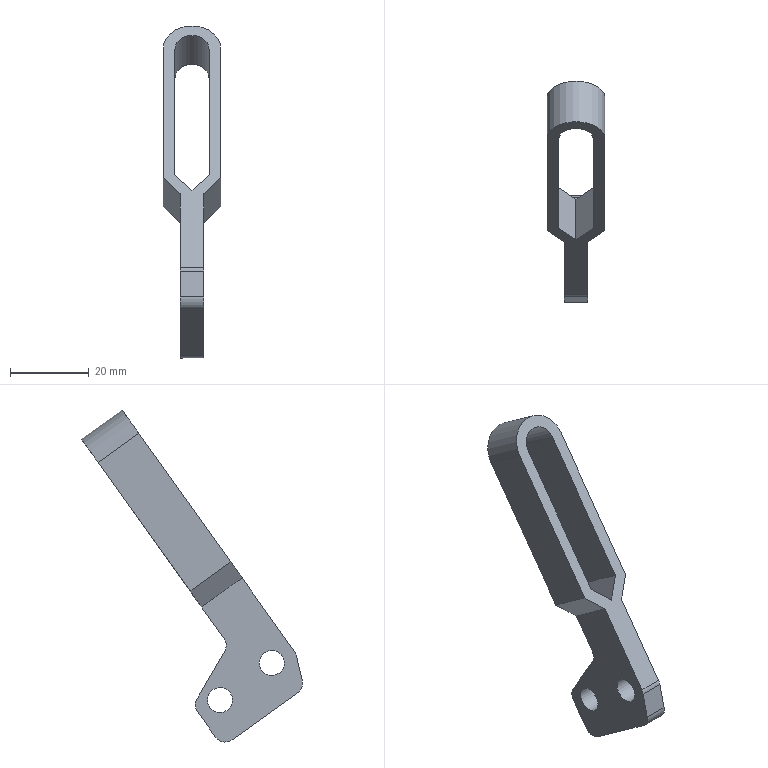Component | SolidWorks | AD12-MC01H-4_2_03.SDASM-1_AD12-_MC01H-4_s.sdprt-1 | 1 solid | 27 faces | box 14.7 x 56.22 x 84.43 mm | volume 7823 mm3 | plane 16 | cylinder 11 | commonest cylinder face diameters 6 x5 6.35 x4 14.7 x1 8.7 x1
STEP:
#1=COLOUR_RGB('',0.7922,0.8196,0.9333);
#2=FILL_AREA_STYLE_COLOUR('',#1);
#3=FILL_AREA_STYLE('',(#2));
#4=SURFACE_STYLE_FILL_AREA(#3);
#5=SURFACE_SIDE_STYLE('',(#4));
#6=SURFACE_STYLE_USAGE(.BOTH.,#5);
#7=PRESENTATION_STYLE_ASSIGNMENT((#6));
#8=CARTESIAN_POINT('',(-12.398,-8.023,13.819));
#9=VERTEX_POINT('',#8);
#10=CARTESIAN_POINT('',(-12.398,-8.168,13.616));
#11=VERTEX_POINT('',#10);
#12=CARTESIAN_POINT('',(-12.398,-8.096,13.717));
#13=DIRECTION('',(1.,0.,0.));
#14=DIRECTION('',(0.,-0.5813,-0.8137));
#15=AXIS2_PLACEMENT_3D('',#12,#13,#14);
#16=CIRCLE('',#15,0.125);
#17=EDGE_CURVE('',#9,#11,#16,.T.);
#18=ORIENTED_EDGE('',*,*,#17,.F.);
#19=CARTESIAN_POINT('',(-12.162,-8.023,13.819));
#20=VERTEX_POINT('',#19);
#21=CARTESIAN_POINT('',(-12.398,-8.023,13.819));
#22=DIRECTION('',(1.,0.,0.));
#23=VECTOR('',#22,39.37);
#24=LINE('',#21,#23);
#25=EDGE_CURVE('',#9,#20,#24,.T.);
#26=ORIENTED_EDGE('',*,*,#25,.T.);
#27=CARTESIAN_POINT('',(-12.162,-8.168,13.616));
#28=VERTEX_POINT('',#27);
#29=CARTESIAN_POINT('',(-12.162,-8.096,13.717));
#30=DIRECTION('',(1.,0.,0.));
#31=DIRECTION('',(0.,-0.5813,-0.8137));
#32=AXIS2_PLACEMENT_3D('',#29,#30,#31);
#33=CIRCLE('',#32,0.125);
#34=EDGE_CURVE('',#20,#28,#33,.T.);
#35=ORIENTED_EDGE('',*,*,#34,.T.);
#36=CARTESIAN_POINT('',(-12.398,-8.168,13.616));
#37=DIRECTION('',(1.,0.,0.));
#38=VECTOR('',#37,39.37);
#39=LINE('',#36,#38);
#40=EDGE_CURVE('',#11,#28,#39,.T.);
#41=ORIENTED_EDGE('',*,*,#40,.F.);
#42=EDGE_LOOP('',(#18,#26,#35,#41));
#43=FACE_OUTER_BOUND('',#42,.T.);
#44=CARTESIAN_POINT('',(-12.398,-8.096,13.717));
#45=DIRECTION('',(1.,0.,0.));
#46=DIRECTION('',(0.,-0.5813,-0.8137));
#47=AXIS2_PLACEMENT_3D('',#44,#45,#46);
#48=CYLINDRICAL_SURFACE('',#47,0.125);
#49=ADVANCED_FACE('',(#43),#48,.F.);
#50=CARTESIAN_POINT('',(-12.398,-8.542,14.19));
#51=VERTEX_POINT('',#50);
#52=CARTESIAN_POINT('',(-12.398,-8.687,13.986));
#53=VERTEX_POINT('',#52);
#54=CARTESIAN_POINT('',(-12.398,-8.615,14.088));
#55=DIRECTION('',(1.,0.,0.));
#56=DIRECTION('',(0.,-0.5813,-0.8137));
#57=AXIS2_PLACEMENT_3D('',#54,#55,#56);
#58=CIRCLE('',#57,0.125);
#59=EDGE_CURVE('',#51,#53,#58,.T.);
#60=ORIENTED_EDGE('',*,*,#59,.F.);
#61=CARTESIAN_POINT('',(-12.162,-8.542,14.19));
#62=VERTEX_POINT('',#61);
#63=CARTESIAN_POINT('',(-12.398,-8.542,14.19));
#64=DIRECTION('',(1.,0.,0.));
#65=VECTOR('',#64,39.37);
#66=LINE('',#63,#65);
#67=EDGE_CURVE('',#51,#62,#66,.T.);
#68=ORIENTED_EDGE('',*,*,#67,.T.);
#69=CARTESIAN_POINT('',(-12.162,-8.687,13.986));
#70=VERTEX_POINT('',#69);
#71=CARTESIAN_POINT('',(-12.162,-8.615,14.088));
#72=DIRECTION('',(1.,0.,0.));
#73=DIRECTION('',(0.,-0.5813,-0.8137));
#74=AXIS2_PLACEMENT_3D('',#71,#72,#73);
#75=CIRCLE('',#74,0.125);
#76=EDGE_CURVE('',#62,#70,#75,.T.);
#77=ORIENTED_EDGE('',*,*,#76,.T.);
#78=CARTESIAN_POINT('',(-12.398,-8.687,13.986));
#79=DIRECTION('',(1.,0.,0.));
#80=VECTOR('',#79,39.37);
#81=LINE('',#78,#80);
#82=EDGE_CURVE('',#53,#70,#81,.T.);
#83=ORIENTED_EDGE('',*,*,#82,.F.);
#84=EDGE_LOOP('',(#60,#68,#77,#83));
#85=FACE_OUTER_BOUND('',#84,.T.);
#86=CARTESIAN_POINT('',(-12.398,-8.615,14.088));
#87=DIRECTION('',(1.,0.,0.));
#88=DIRECTION('',(0.,-0.5813,-0.8137));
#89=AXIS2_PLACEMENT_3D('',#86,#87,#88);
#90=CYLINDRICAL_SURFACE('',#89,0.125);
#91=ADVANCED_FACE('',(#85),#90,.F.);
#92=CARTESIAN_POINT('',(-12.162,-8.096,13.717));
#93=DIRECTION('',(1.,0.,0.));
#94=DIRECTION('',(0.,-0.5813,-0.8137));
#95=AXIS2_PLACEMENT_3D('',#92,#93,#94);
#96=CIRCLE('',#95,0.125);
#97=EDGE_CURVE('',#28,#20,#96,.T.);
#98=ORIENTED_EDGE('',*,*,#97,.F.);
#99=ORIENTED_EDGE('',*,*,#34,.F.);
#100=EDGE_LOOP('',(#98,#99));
#101=FACE_BOUND('',#100,.T.);
#102=CARTESIAN_POINT('',(-12.162,-7.91,14.648));
#103=VERTEX_POINT('',#102);
#104=CARTESIAN_POINT('',(-12.162,-8.136,14.331));
#105=VERTEX_POINT('',#104);
#106=CARTESIAN_POINT('',(-12.162,-7.91,14.648));
#107=DIRECTION('',(0.,-0.5813,-0.8137));
#108=VECTOR('',#107,39.37);
#109=LINE('',#106,#108);
#110=EDGE_CURVE('',#103,#105,#109,.T.);
#111=ORIENTED_EDGE('',*,*,#110,.F.);
#112=CARTESIAN_POINT('',(-12.162,-8.316,14.939));
#113=VERTEX_POINT('',#112);
#114=CARTESIAN_POINT('',(-12.162,-7.195,14.138));
#115=DIRECTION('',(0.,0.8137,-0.5813));
#116=VECTOR('',#115,39.37);
#117=LINE('',#114,#116);
#118=EDGE_CURVE('',#113,#103,#117,.T.);
#119=ORIENTED_EDGE('',*,*,#118,.F.);
#120=CARTESIAN_POINT('',(-12.162,-8.84,14.206));
#121=VERTEX_POINT('',#120);
#122=CARTESIAN_POINT('',(-12.162,-8.316,14.939));
#123=DIRECTION('',(0.,0.5813,0.8137));
#124=VECTOR('',#123,39.37);
#125=LINE('',#122,#124);
#126=EDGE_CURVE('',#121,#113,#125,.T.);
#127=ORIENTED_EDGE('',*,*,#126,.F.);
#128=CARTESIAN_POINT('',(-12.162,-8.859,14.164));
#129=VERTEX_POINT('',#128);
#130=CARTESIAN_POINT('',(-12.162,-8.744,14.137));
#131=DIRECTION('',(-1.,0.,0.));
#132=DIRECTION('',(0.,-0.5813,-0.8137));
#133=AXIS2_PLACEMENT_3D('',#130,#131,#132);
#134=CIRCLE('',#133,0.1181);
#135=EDGE_CURVE('',#129,#121,#134,.T.);
#136=ORIENTED_EDGE('',*,*,#135,.F.);
#137=CARTESIAN_POINT('',(-12.162,-8.918,13.911));
#138=VERTEX_POINT('',#137);
#139=CARTESIAN_POINT('',(-12.162,-8.918,13.911));
#140=DIRECTION('',(0.,0.2274,0.9738));
#141=VECTOR('',#140,39.37);
#142=LINE('',#139,#141);
#143=EDGE_CURVE('',#138,#129,#142,.T.);
#144=ORIENTED_EDGE('',*,*,#143,.F.);
#145=CARTESIAN_POINT('',(-12.162,-8.872,13.788));
#146=VERTEX_POINT('',#145);
#147=CARTESIAN_POINT('',(-12.162,-8.803,13.884));
#148=DIRECTION('',(-1.,0.,0.));
#149=DIRECTION('',(0.,-0.5813,-0.8137));
#150=AXIS2_PLACEMENT_3D('',#147,#148,#149);
#151=CIRCLE('',#150,0.1181);
#152=EDGE_CURVE('',#146,#138,#151,.T.);
#153=ORIENTED_EDGE('',*,*,#152,.F.);
#154=CARTESIAN_POINT('',(-12.162,-8.216,13.319));
#155=VERTEX_POINT('',#154);
#156=CARTESIAN_POINT('',(-12.162,-7.927,13.113));
#157=DIRECTION('',(0.,-0.8137,0.5813));
#158=VECTOR('',#157,39.37);
#159=LINE('',#156,#158);
#160=EDGE_CURVE('',#155,#146,#159,.T.);
#161=ORIENTED_EDGE('',*,*,#160,.F.);
#162=CARTESIAN_POINT('',(-12.162,-8.051,13.347));
#163=VERTEX_POINT('',#162);
#164=CARTESIAN_POINT('',(-12.162,-8.147,13.415));
#165=DIRECTION('',(-1.,0.,0.));
#166=DIRECTION('',(0.,-0.5813,-0.8137));
#167=AXIS2_PLACEMENT_3D('',#164,#165,#166);
#168=CIRCLE('',#167,0.1181);
#169=EDGE_CURVE('',#163,#155,#168,.T.);
#170=ORIENTED_EDGE('',*,*,#169,.F.);
#171=CARTESIAN_POINT('',(-12.162,-7.87,13.599));
#172=VERTEX_POINT('',#171);
#173=CARTESIAN_POINT('',(-12.162,-7.387,14.275));
#174=DIRECTION('',(0.,-0.5813,-0.8137));
#175=VECTOR('',#174,39.37);
#176=LINE('',#173,#175);
#177=EDGE_CURVE('',#172,#163,#176,.T.);
#178=ORIENTED_EDGE('',*,*,#177,.F.);
#179=CARTESIAN_POINT('',(-12.162,-7.865,13.727));
#180=VERTEX_POINT('',#179);
#181=CARTESIAN_POINT('',(-12.162,-7.967,13.668));
#182=DIRECTION('',(-1.,0.,0.));
#183=DIRECTION('',(0.,-0.5813,-0.8137));
#184=AXIS2_PLACEMENT_3D('',#181,#182,#183);
#185=CIRCLE('',#184,0.1181);
#186=EDGE_CURVE('',#180,#172,#185,.T.);
#187=ORIENTED_EDGE('',*,*,#186,.F.);
#188=CARTESIAN_POINT('',(-12.162,-8.142,14.203));
#189=VERTEX_POINT('',#188);
#190=CARTESIAN_POINT('',(-12.162,-8.142,14.203));
#191=DIRECTION('',(0.,0.5037,-0.8639));
#192=VECTOR('',#191,39.37);
#193=LINE('',#190,#192);
#194=EDGE_CURVE('',#189,#180,#193,.T.);
#195=ORIENTED_EDGE('',*,*,#194,.F.);
#196=CARTESIAN_POINT('',(-12.162,-8.04,14.263));
#197=DIRECTION('',(1.,0.,0.));
#198=DIRECTION('',(0.,-0.5813,-0.8137));
#199=AXIS2_PLACEMENT_3D('',#196,#197,#198);
#200=CIRCLE('',#199,0.1181);
#201=EDGE_CURVE('',#105,#189,#200,.T.);
#202=ORIENTED_EDGE('',*,*,#201,.F.);
#203=EDGE_LOOP('',(#111,#119,#127,#136,#144,#153,#161,#170,#178,#187,#195,#202));
#204=FACE_OUTER_BOUND('',#203,.T.);
#205=CARTESIAN_POINT('',(-12.162,-8.615,14.088));
#206=DIRECTION('',(1.,0.,0.));
#207=DIRECTION('',(0.,-0.5813,-0.8137));
#208=AXIS2_PLACEMENT_3D('',#205,#206,#207);
#209=CIRCLE('',#208,0.125);
#210=EDGE_CURVE('',#70,#62,#209,.T.);
#211=ORIENTED_EDGE('',*,*,#210,.F.);
#212=ORIENTED_EDGE('',*,*,#76,.F.);
#213=EDGE_LOOP('',(#211,#212));
#214=FACE_BOUND('',#213,.T.);
#215=CARTESIAN_POINT('',(-12.162,-7.195,14.138));
#216=DIRECTION('',(-1.,0.,0.));
#217=DIRECTION('',(0.,0.5813,0.8137));
#218=AXIS2_PLACEMENT_3D('',#215,#216,#217);
#219=PLANE('',#218);
#220=ADVANCED_FACE('',(#101,#204,#214),#219,.F.);
#221=ORIENTED_EDGE('',*,*,#25,.F.);
#222=CARTESIAN_POINT('',(-12.398,-8.096,13.717));
#223=DIRECTION('',(1.,0.,0.));
#224=DIRECTION('',(0.,-0.5813,-0.8137));
#225=AXIS2_PLACEMENT_3D('',#222,#223,#224);
#226=CIRCLE('',#225,0.125);
#227=EDGE_CURVE('',#11,#9,#226,.T.);
#228=ORIENTED_EDGE('',*,*,#227,.F.);
#229=ORIENTED_EDGE('',*,*,#40,.T.);
#230=ORIENTED_EDGE('',*,*,#97,.T.);
#231=EDGE_LOOP('',(#221,#228,#229,#230));
#232=FACE_OUTER_BOUND('',#231,.T.);
#233=CARTESIAN_POINT('',(-12.398,-8.096,13.717));
#234=DIRECTION('',(1.,0.,0.));
#235=DIRECTION('',(0.,-0.5813,-0.8137));
#236=AXIS2_PLACEMENT_3D('',#233,#234,#235);
#237=CYLINDRICAL_SURFACE('',#236,0.125);
#238=ADVANCED_FACE('',(#232),#237,.F.);
#239=CARTESIAN_POINT('',(-12.398,-8.142,14.203));
#240=VERTEX_POINT('',#239);
#241=CARTESIAN_POINT('',(-10.902,-8.142,14.203));
#242=DIRECTION('',(1.,0.,0.));
#243=VECTOR('',#242,39.37);
#244=LINE('',#241,#243);
#245=EDGE_CURVE('',#240,#189,#244,.T.);
#246=ORIENTED_EDGE('',*,*,#245,.F.);
#247=CARTESIAN_POINT('',(-12.398,-8.136,14.331));
#248=VERTEX_POINT('',#247);
#249=CARTESIAN_POINT('',(-12.398,-8.04,14.263));
#250=DIRECTION('',(1.,0.,0.));
#251=DIRECTION('',(0.,-0.5813,-0.8137));
#252=AXIS2_PLACEMENT_3D('',#249,#250,#251);
#253=CIRCLE('',#252,0.1181);
#254=EDGE_CURVE('',#248,#240,#253,.T.);
#255=ORIENTED_EDGE('',*,*,#254,.F.);
#256=CARTESIAN_POINT('',(-10.902,-8.136,14.331));
#257=DIRECTION('',(-1.,0.,0.));
#258=VECTOR('',#257,39.37);
#259=LINE('',#256,#258);
#260=EDGE_CURVE('',#105,#248,#259,.T.);
#261=ORIENTED_EDGE('',*,*,#260,.F.);
#262=ORIENTED_EDGE('',*,*,#201,.T.);
#263=EDGE_LOOP('',(#246,#255,#261,#262));
#264=FACE_OUTER_BOUND('',#263,.T.);
#265=CARTESIAN_POINT('',(-10.902,-8.04,14.263));
#266=DIRECTION('',(1.,0.,0.));
#267=DIRECTION('',(0.,-0.5813,-0.8137));
#268=AXIS2_PLACEMENT_3D('',#265,#266,#267);
#269=CYLINDRICAL_SURFACE('',#268,0.1181);
#270=ADVANCED_FACE('',(#264),#269,.F.);
#271=CARTESIAN_POINT('',(-12.398,-7.91,14.648));
#272=VERTEX_POINT('',#271);
#273=CARTESIAN_POINT('',(-12.398,-8.136,14.331));
#274=DIRECTION('',(0.,-0.5813,-0.8137));
#275=VECTOR('',#274,39.37);
#276=LINE('',#273,#275);
#277=EDGE_CURVE('',#272,#248,#276,.T.);
#278=ORIENTED_EDGE('',*,*,#277,.F.);
#279=CARTESIAN_POINT('',(-12.569,-7.795,14.809));
#280=VERTEX_POINT('',#279);
#281=CARTESIAN_POINT('',(-12.569,-7.795,14.809));
#282=DIRECTION('',(0.6555,-0.439,-0.6145));
#283=VECTOR('',#282,39.37);
#284=LINE('',#281,#283);
#285=EDGE_CURVE('',#280,#272,#284,.T.);
#286=ORIENTED_EDGE('',*,*,#285,.F.);
#287=CARTESIAN_POINT('',(-12.569,-6.876,16.095));
#288=VERTEX_POINT('',#287);
#289=CARTESIAN_POINT('',(-12.569,-8.136,14.331));
#290=DIRECTION('',(0.,-0.5813,-0.8137));
#291=VECTOR('',#290,39.37);
#292=LINE('',#289,#291);
#293=EDGE_CURVE('',#288,#280,#292,.T.);
#294=ORIENTED_EDGE('',*,*,#293,.F.);
#295=CARTESIAN_POINT('',(-11.991,-6.876,16.095));
#296=VERTEX_POINT('',#295);
#297=CARTESIAN_POINT('',(-12.28,-6.876,16.095));
#298=DIRECTION('',(0.,-0.8137,0.5813));
#299=DIRECTION('',(1.,0.,0.));
#300=AXIS2_PLACEMENT_3D('',#297,#298,#299);
#301=CIRCLE('',#300,0.2894);
#302=EDGE_CURVE('',#296,#288,#301,.T.);
#303=ORIENTED_EDGE('',*,*,#302,.F.);
#304=CARTESIAN_POINT('',(-11.991,-7.795,14.809));
#305=VERTEX_POINT('',#304);
#306=CARTESIAN_POINT('',(-11.991,-8.136,14.331));
#307=DIRECTION('',(0.,0.5813,0.8137));
#308=VECTOR('',#307,39.37);
#309=LINE('',#306,#308);
#310=EDGE_CURVE('',#305,#296,#309,.T.);
#311=ORIENTED_EDGE('',*,*,#310,.F.);
#312=CARTESIAN_POINT('',(-12.162,-7.91,14.648));
#313=DIRECTION('',(0.6555,0.439,0.6145));
#314=VECTOR('',#313,39.37);
#315=LINE('',#312,#314);
#316=EDGE_CURVE('',#103,#305,#315,.T.);
#317=ORIENTED_EDGE('',*,*,#316,.F.);
#318=ORIENTED_EDGE('',*,*,#110,.T.);
#319=ORIENTED_EDGE('',*,*,#260,.T.);
#320=EDGE_LOOP('',(#278,#286,#294,#303,#311,#317,#318,#319));
#321=FACE_OUTER_BOUND('',#320,.T.);
#322=CARTESIAN_POINT('',(-12.28,-7.885,14.683));
#323=VERTEX_POINT('',#322);
#324=CARTESIAN_POINT('',(-12.451,-7.771,14.842));
#325=VERTEX_POINT('',#324);
#326=CARTESIAN_POINT('',(-12.28,-7.885,14.683));
#327=DIRECTION('',(-0.6577,0.4379,0.6129));
#328=VECTOR('',#327,39.37);
#329=LINE('',#326,#328);
#330=EDGE_CURVE('',#323,#325,#329,.T.);
#331=ORIENTED_EDGE('',*,*,#330,.F.);
#332=CARTESIAN_POINT('',(-12.109,-7.771,14.842));
#333=VERTEX_POINT('',#332);
#334=CARTESIAN_POINT('',(-12.109,-7.771,14.842));
#335=DIRECTION('',(-0.6577,-0.4379,-0.6129));
#336=VECTOR('',#335,39.37);
#337=LINE('',#334,#336);
#338=EDGE_CURVE('',#333,#323,#337,.T.);
#339=ORIENTED_EDGE('',*,*,#338,.F.);
#340=CARTESIAN_POINT('',(-12.109,-6.876,16.095));
#341=VERTEX_POINT('',#340);
#342=CARTESIAN_POINT('',(-12.109,-8.136,14.331));
#343=DIRECTION('',(0.,-0.5813,-0.8137));
#344=VECTOR('',#343,39.37);
#345=LINE('',#342,#344);
#346=EDGE_CURVE('',#341,#333,#345,.T.);
#347=ORIENTED_EDGE('',*,*,#346,.F.);
#348=CARTESIAN_POINT('',(-12.451,-6.876,16.095));
#349=VERTEX_POINT('',#348);
#350=CARTESIAN_POINT('',(-12.28,-6.876,16.095));
#351=DIRECTION('',(0.,0.8137,-0.5813));
#352=DIRECTION('',(1.,0.,0.));
#353=AXIS2_PLACEMENT_3D('',#350,#351,#352);
#354=CIRCLE('',#353,0.1713);
#355=EDGE_CURVE('',#349,#341,#354,.T.);
#356=ORIENTED_EDGE('',*,*,#355,.F.);
#357=CARTESIAN_POINT('',(-12.451,-8.136,14.331));
#358=DIRECTION('',(0.,0.5813,0.8137));
#359=VECTOR('',#358,39.37);
#360=LINE('',#357,#359);
#361=EDGE_CURVE('',#325,#349,#360,.T.);
#362=ORIENTED_EDGE('',*,*,#361,.F.);
#363=EDGE_LOOP('',(#331,#339,#347,#356,#362));
#364=FACE_BOUND('',#363,.T.);
#365=CARTESIAN_POINT('',(-10.902,-8.136,14.331));
#366=DIRECTION('',(0.,-0.8137,0.5813));
#367=DIRECTION('',(-1.,0.,0.));
#368=AXIS2_PLACEMENT_3D('',#365,#366,#367);
#369=PLANE('',#368);
#370=ADVANCED_FACE('',(#321,#364),#369,.F.);
#371=ORIENTED_EDGE('',*,*,#316,.T.);
#372=CARTESIAN_POINT('',(-11.991,-8.202,15.099));
#373=VERTEX_POINT('',#372);
#374=CARTESIAN_POINT('',(-11.991,-7.08,14.299));
#375=DIRECTION('',(0.,0.8137,-0.5813));
#376=VECTOR('',#375,39.37);
#377=LINE('',#374,#376);
#378=EDGE_CURVE('',#373,#305,#377,.T.);
#379=ORIENTED_EDGE('',*,*,#378,.F.);
#380=CARTESIAN_POINT('',(-11.991,-8.202,15.099));
#381=DIRECTION('',(0.6555,0.439,0.6145));
#382=VECTOR('',#381,39.37);
#383=LINE('',#380,#382);
#384=EDGE_CURVE('',#113,#373,#383,.T.);
#385=ORIENTED_EDGE('',*,*,#384,.F.);
#386=ORIENTED_EDGE('',*,*,#118,.T.);
#387=EDGE_LOOP('',(#371,#379,#385,#386));
#388=FACE_OUTER_BOUND('',#387,.T.);
#389=CARTESIAN_POINT('',(-11.991,-7.08,14.299));
#390=DIRECTION('',(-0.7552,0.381,0.5334));
#391=DIRECTION('',(0.6555,0.439,0.6145));
#392=AXIS2_PLACEMENT_3D('',#389,#390,#391);
#393=PLANE('',#392);
#394=ADVANCED_FACE('',(#388),#393,.F.);
#395=CARTESIAN_POINT('',(-12.398,-8.84,14.206));
#396=VERTEX_POINT('',#395);
#397=CARTESIAN_POINT('',(-12.28,-8.84,14.206));
#398=DIRECTION('',(-1.,0.,0.));
#399=VECTOR('',#398,39.37);
#400=LINE('',#397,#399);
#401=EDGE_CURVE('',#121,#396,#400,.T.);
#402=ORIENTED_EDGE('',*,*,#401,.F.);
#403=ORIENTED_EDGE('',*,*,#126,.T.);
#404=ORIENTED_EDGE('',*,*,#384,.T.);
#405=CARTESIAN_POINT('',(-11.991,-7.283,16.386));
#406=VERTEX_POINT('',#405);
#407=CARTESIAN_POINT('',(-11.991,-7.283,16.386));
#408=DIRECTION('',(0.,-0.5813,-0.8137));
#409=VECTOR('',#408,39.37);
#410=LINE('',#407,#409);
#411=EDGE_CURVE('',#406,#373,#410,.T.);
#412=ORIENTED_EDGE('',*,*,#411,.F.);
#413=CARTESIAN_POINT('',(-12.569,-7.283,16.386));
#414=VERTEX_POINT('',#413);
#415=CARTESIAN_POINT('',(-12.28,-7.283,16.386));
#416=DIRECTION('',(0.,0.8137,-0.5813));
#417=DIRECTION('',(1.,0.,0.));
#418=AXIS2_PLACEMENT_3D('',#415,#416,#417);
#419=CIRCLE('',#418,0.2894);
#420=EDGE_CURVE('',#414,#406,#419,.T.);
#421=ORIENTED_EDGE('',*,*,#420,.F.);
#422=CARTESIAN_POINT('',(-12.569,-8.202,15.099));
#423=VERTEX_POINT('',#422);
#424=CARTESIAN_POINT('',(-12.569,-7.283,16.386));
#425=DIRECTION('',(0.,0.5813,0.8137));
#426=VECTOR('',#425,39.37);
#427=LINE('',#424,#426);
#428=EDGE_CURVE('',#423,#414,#427,.T.);
#429=ORIENTED_EDGE('',*,*,#428,.F.);
#430=CARTESIAN_POINT('',(-12.398,-8.316,14.939));
#431=VERTEX_POINT('',#430);
#432=CARTESIAN_POINT('',(-12.398,-8.316,14.939));
#433=DIRECTION('',(-0.6555,0.439,0.6145));
#434=VECTOR('',#433,39.37);
#435=LINE('',#432,#434);
#436=EDGE_CURVE('',#431,#423,#435,.T.);
#437=ORIENTED_EDGE('',*,*,#436,.F.);
#438=CARTESIAN_POINT('',(-12.398,-7.283,16.386));
#439=DIRECTION('',(0.,0.5813,0.8137));
#440=VECTOR('',#439,39.37);
#441=LINE('',#438,#440);
#442=EDGE_CURVE('',#396,#431,#441,.T.);
#443=ORIENTED_EDGE('',*,*,#442,.F.);
#444=EDGE_LOOP('',(#402,#403,#404,#412,#421,#429,#437,#443));
#445=FACE_OUTER_BOUND('',#444,.T.);
#446=CARTESIAN_POINT('',(-12.109,-7.283,16.386));
#447=VERTEX_POINT('',#446);
#448=CARTESIAN_POINT('',(-12.451,-7.283,16.386));
#449=VERTEX_POINT('',#448);
#450=CARTESIAN_POINT('',(-12.28,-7.283,16.386));
#451=DIRECTION('',(0.,-0.8137,0.5813));
#452=DIRECTION('',(1.,0.,0.));
#453=AXIS2_PLACEMENT_3D('',#450,#451,#452);
#454=CIRCLE('',#453,0.1713);
#455=EDGE_CURVE('',#447,#449,#454,.T.);
#456=ORIENTED_EDGE('',*,*,#455,.F.);
#457=CARTESIAN_POINT('',(-12.109,-8.178,15.133));
#458=VERTEX_POINT('',#457);
#459=CARTESIAN_POINT('',(-12.109,-7.283,16.386));
#460=DIRECTION('',(0.,0.5813,0.8137));
#461=VECTOR('',#460,39.37);
#462=LINE('',#459,#461);
#463=EDGE_CURVE('',#458,#447,#462,.T.);
#464=ORIENTED_EDGE('',*,*,#463,.F.);
#465=CARTESIAN_POINT('',(-12.28,-8.292,14.973));
#466=VERTEX_POINT('',#465);
#467=CARTESIAN_POINT('',(-12.28,-8.292,14.973));
#468=DIRECTION('',(0.6577,0.4379,0.6129));
#469=VECTOR('',#468,39.37);
#470=LINE('',#467,#469);
#471=EDGE_CURVE('',#466,#458,#470,.T.);
#472=ORIENTED_EDGE('',*,*,#471,.F.);
#473=CARTESIAN_POINT('',(-12.451,-8.178,15.133));
#474=VERTEX_POINT('',#473);
#475=CARTESIAN_POINT('',(-12.451,-8.178,15.133));
#476=DIRECTION('',(0.6577,-0.4379,-0.6129));
#477=VECTOR('',#476,39.37);
#478=LINE('',#475,#477);
#479=EDGE_CURVE('',#474,#466,#478,.T.);
#480=ORIENTED_EDGE('',*,*,#479,.F.);
#481=CARTESIAN_POINT('',(-12.451,-7.283,16.386));
#482=DIRECTION('',(0.,-0.5813,-0.8137));
#483=VECTOR('',#482,39.37);
#484=LINE('',#481,#483);
#485=EDGE_CURVE('',#449,#474,#484,.T.);
#486=ORIENTED_EDGE('',*,*,#485,.F.);
#487=EDGE_LOOP('',(#456,#464,#472,#480,#486));
#488=FACE_BOUND('',#487,.T.);
#489=CARTESIAN_POINT('',(-12.28,-7.283,16.386));
#490=DIRECTION('',(0.,0.8137,-0.5813));
#491=DIRECTION('',(1.,0.,0.));
#492=AXIS2_PLACEMENT_3D('',#489,#490,#491);
#493=PLANE('',#492);
#494=ADVANCED_FACE('',(#445,#488),#493,.F.);
#495=CARTESIAN_POINT('',(-12.398,-8.918,13.911));
#496=VERTEX_POINT('',#495);
#497=CARTESIAN_POINT('',(-12.398,-8.859,14.164));
#498=VERTEX_POINT('',#497);
#499=CARTESIAN_POINT('',(-12.398,-8.859,14.164));
#500=DIRECTION('',(0.,0.2274,0.9738));
#501=VECTOR('',#500,39.37);
#502=LINE('',#499,#501);
#503=EDGE_CURVE('',#496,#498,#502,.T.);
#504=ORIENTED_EDGE('',*,*,#503,.F.);
#505=CARTESIAN_POINT('',(-10.902,-8.918,13.911));
#506=DIRECTION('',(-1.,0.,0.));
#507=VECTOR('',#506,39.37);
#508=LINE('',#505,#507);
#509=EDGE_CURVE('',#138,#496,#508,.T.);
#510=ORIENTED_EDGE('',*,*,#509,.F.);
#511=ORIENTED_EDGE('',*,*,#143,.T.);
#512=CARTESIAN_POINT('',(-10.902,-8.859,14.164));
#513=DIRECTION('',(1.,0.,0.));
#514=VECTOR('',#513,39.37);
#515=LINE('',#512,#514);
#516=EDGE_CURVE('',#498,#129,#515,.T.);
#517=ORIENTED_EDGE('',*,*,#516,.F.);
#518=EDGE_LOOP('',(#504,#510,#511,#517));
#519=FACE_OUTER_BOUND('',#518,.T.);
#520=CARTESIAN_POINT('',(-10.902,-8.859,14.164));
#521=DIRECTION('',(0.,0.9738,-0.2274));
#522=DIRECTION('',(0.,0.2274,0.9738));
#523=AXIS2_PLACEMENT_3D('',#520,#521,#522);
#524=PLANE('',#523);
#525=ADVANCED_FACE('',(#519),#524,.F.);
#526=CARTESIAN_POINT('',(-12.398,-8.872,13.788));
#527=VERTEX_POINT('',#526);
#528=CARTESIAN_POINT('',(-10.902,-8.872,13.788));
#529=DIRECTION('',(1.,0.,0.));
#530=VECTOR('',#529,39.37);
#531=LINE('',#528,#530);
#532=EDGE_CURVE('',#527,#146,#531,.T.);
#533=ORIENTED_EDGE('',*,*,#532,.T.);
#534=ORIENTED_EDGE('',*,*,#152,.T.);
#535=ORIENTED_EDGE('',*,*,#509,.T.);
#536=CARTESIAN_POINT('',(-12.398,-8.803,13.884));
#537=DIRECTION('',(1.,0.,0.));
#538=DIRECTION('',(0.,-0.5813,-0.8137));
#539=AXIS2_PLACEMENT_3D('',#536,#537,#538);
#540=CIRCLE('',#539,0.1181);
#541=EDGE_CURVE('',#496,#527,#540,.T.);
#542=ORIENTED_EDGE('',*,*,#541,.T.);
#543=EDGE_LOOP('',(#533,#534,#535,#542));
#544=FACE_OUTER_BOUND('',#543,.T.);
#545=CARTESIAN_POINT('',(-10.902,-8.803,13.884));
#546=DIRECTION('',(1.,0.,0.));
#547=DIRECTION('',(0.,-0.5813,-0.8137));
#548=AXIS2_PLACEMENT_3D('',#545,#546,#547);
#549=CYLINDRICAL_SURFACE('',#548,0.1181);
#550=ADVANCED_FACE('',(#544),#549,.T.);
#551=CARTESIAN_POINT('',(-12.398,-8.216,13.319));
#552=VERTEX_POINT('',#551);
#553=CARTESIAN_POINT('',(-12.398,-8.872,13.788));
#554=DIRECTION('',(0.,-0.8137,0.5813));
#555=VECTOR('',#554,39.37);
#556=LINE('',#553,#555);
#557=EDGE_CURVE('',#552,#527,#556,.T.);
#558=ORIENTED_EDGE('',*,*,#557,.F.);
#559=CARTESIAN_POINT('',(-10.902,-8.216,13.319));
#560=DIRECTION('',(-1.,0.,0.));
#561=VECTOR('',#560,39.37);
#562=LINE('',#559,#561);
#563=EDGE_CURVE('',#155,#552,#562,.T.);
#564=ORIENTED_EDGE('',*,*,#563,.F.);
#565=ORIENTED_EDGE('',*,*,#160,.T.);
#566=ORIENTED_EDGE('',*,*,#532,.F.);
#567=EDGE_LOOP('',(#558,#564,#565,#566));
#568=FACE_OUTER_BOUND('',#567,.T.);
#569=CARTESIAN_POINT('',(-10.902,-8.872,13.788));
#570=DIRECTION('',(0.,0.5813,0.8137));
#571=DIRECTION('',(1.,0.,0.));
#572=AXIS2_PLACEMENT_3D('',#569,#570,#571);
#573=PLANE('',#572);
#574=ADVANCED_FACE('',(#568),#573,.F.);
#575=CARTESIAN_POINT('',(-12.398,-8.051,13.347));
#576=VERTEX_POINT('',#575);
#577=CARTESIAN_POINT('',(-10.902,-8.051,13.347));
#578=DIRECTION('',(1.,0.,0.));
#579=VECTOR('',#578,39.37);
#580=LINE('',#577,#579);
#581=EDGE_CURVE('',#576,#163,#580,.T.);
#582=ORIENTED_EDGE('',*,*,#581,.T.);
#583=ORIENTED_EDGE('',*,*,#169,.T.);
#584=ORIENTED_EDGE('',*,*,#563,.T.);
#585=CARTESIAN_POINT('',(-12.398,-8.147,13.415));
#586=DIRECTION('',(1.,0.,0.));
#587=DIRECTION('',(0.,-0.5813,-0.8137));
#588=AXIS2_PLACEMENT_3D('',#585,#586,#587);
#589=CIRCLE('',#588,0.1181);
#590=EDGE_CURVE('',#552,#576,#589,.T.);
#591=ORIENTED_EDGE('',*,*,#590,.T.);
#592=EDGE_LOOP('',(#582,#583,#584,#591));
#593=FACE_OUTER_BOUND('',#592,.T.);
#594=CARTESIAN_POINT('',(-10.902,-8.147,13.415));
#595=DIRECTION('',(1.,0.,0.));
#596=DIRECTION('',(0.,-0.5813,-0.8137));
#597=AXIS2_PLACEMENT_3D('',#594,#595,#596);
#598=CYLINDRICAL_SURFACE('',#597,0.1181);
#599=ADVANCED_FACE('',(#593),#598,.T.);
#600=CARTESIAN_POINT('',(-12.398,-7.87,13.599));
#601=VERTEX_POINT('',#600);
#602=CARTESIAN_POINT('',(-12.398,-8.051,13.347));
#603=DIRECTION('',(0.,-0.5813,-0.8137));
#604=VECTOR('',#603,39.37);
#605=LINE('',#602,#604);
#606=EDGE_CURVE('',#601,#576,#605,.T.);
#607=ORIENTED_EDGE('',*,*,#606,.F.);
#608=CARTESIAN_POINT('',(-10.902,-7.87,13.599));
#609=DIRECTION('',(-1.,0.,0.));
#610=VECTOR('',#609,39.37);
#611=LINE('',#608,#610);
#612=EDGE_CURVE('',#172,#601,#611,.T.);
#613=ORIENTED_EDGE('',*,*,#612,.F.);
#614=ORIENTED_EDGE('',*,*,#177,.T.);
#615=ORIENTED_EDGE('',*,*,#581,.F.);
#616=EDGE_LOOP('',(#607,#613,#614,#615));
#617=FACE_OUTER_BOUND('',#616,.T.);
#618=CARTESIAN_POINT('',(-10.902,-8.051,13.347));
#619=DIRECTION('',(0.,-0.8137,0.5813));
#620=DIRECTION('',(-1.,0.,0.));
#621=AXIS2_PLACEMENT_3D('',#618,#619,#620);
#622=PLANE('',#621);
#623=ADVANCED_FACE('',(#617),#622,.F.);
#624=CARTESIAN_POINT('',(-12.398,-7.865,13.727));
#625=VERTEX_POINT('',#624);
#626=CARTESIAN_POINT('',(-10.902,-7.865,13.727));
#627=DIRECTION('',(1.,0.,0.));
#628=VECTOR('',#627,39.37);
#629=LINE('',#626,#628);
#630=EDGE_CURVE('',#625,#180,#629,.T.);
#631=ORIENTED_EDGE('',*,*,#630,.T.);
#632=ORIENTED_EDGE('',*,*,#186,.T.);
#633=ORIENTED_EDGE('',*,*,#612,.T.);
#634=CARTESIAN_POINT('',(-12.398,-7.967,13.668));
#635=DIRECTION('',(1.,0.,0.));
#636=DIRECTION('',(0.,-0.5813,-0.8137));
#637=AXIS2_PLACEMENT_3D('',#634,#635,#636);
#638=CIRCLE('',#637,0.1181);
#639=EDGE_CURVE('',#601,#625,#638,.T.);
#640=ORIENTED_EDGE('',*,*,#639,.T.);
#641=EDGE_LOOP('',(#631,#632,#633,#640));
#642=FACE_OUTER_BOUND('',#641,.T.);
#643=CARTESIAN_POINT('',(-10.902,-7.967,13.668));
#644=DIRECTION('',(1.,0.,0.));
#645=DIRECTION('',(0.,-0.5813,-0.8137));
#646=AXIS2_PLACEMENT_3D('',#643,#644,#645);
#647=CYLINDRICAL_SURFACE('',#646,0.1181);
#648=ADVANCED_FACE('',(#642),#647,.T.);
#649=CARTESIAN_POINT('',(-12.398,-7.865,13.727));
#650=DIRECTION('',(0.,0.5037,-0.8639));
#651=VECTOR('',#650,39.37);
#652=LINE('',#649,#651);
#653=EDGE_CURVE('',#240,#625,#652,.T.);
#654=ORIENTED_EDGE('',*,*,#653,.F.);
#655=ORIENTED_EDGE('',*,*,#245,.T.);
#656=ORIENTED_EDGE('',*,*,#194,.T.);
#657=ORIENTED_EDGE('',*,*,#630,.F.);
#658=EDGE_LOOP('',(#654,#655,#656,#657));
#659=FACE_OUTER_BOUND('',#658,.T.);
#660=CARTESIAN_POINT('',(-10.902,-7.865,13.727));
#661=DIRECTION('',(0.,-0.8639,-0.5037));
#662=DIRECTION('',(0.,0.5037,-0.8639));
#663=AXIS2_PLACEMENT_3D('',#660,#661,#662);
#664=PLANE('',#663);
#665=ADVANCED_FACE('',(#659),#664,.F.);
#666=ORIENTED_EDGE('',*,*,#67,.F.);
#667=CARTESIAN_POINT('',(-12.398,-8.615,14.088));
#668=DIRECTION('',(1.,0.,0.));
#669=DIRECTION('',(0.,-0.5813,-0.8137));
#670=AXIS2_PLACEMENT_3D('',#667,#668,#669);
#671=CIRCLE('',#670,0.125);
#672=EDGE_CURVE('',#53,#51,#671,.T.);
#673=ORIENTED_EDGE('',*,*,#672,.F.);
#674=ORIENTED_EDGE('',*,*,#82,.T.);
#675=ORIENTED_EDGE('',*,*,#210,.T.);
#676=EDGE_LOOP('',(#666,#673,#674,#675));
#677=FACE_OUTER_BOUND('',#676,.T.);
#678=CARTESIAN_POINT('',(-12.398,-8.615,14.088));
#679=DIRECTION('',(1.,0.,0.));
#680=DIRECTION('',(0.,-0.5813,-0.8137));
#681=AXIS2_PLACEMENT_3D('',#678,#679,#680);
#682=CYLINDRICAL_SURFACE('',#681,0.125);
#683=ADVANCED_FACE('',(#677),#682,.F.);
#684=ORIENTED_EDGE('',*,*,#227,.T.);
#685=ORIENTED_EDGE('',*,*,#17,.T.);
#686=EDGE_LOOP('',(#684,#685));
#687=FACE_BOUND('',#686,.T.);
#688=ORIENTED_EDGE('',*,*,#277,.T.);
#689=ORIENTED_EDGE('',*,*,#254,.T.);
#690=ORIENTED_EDGE('',*,*,#653,.T.);
#691=ORIENTED_EDGE('',*,*,#639,.F.);
#692=ORIENTED_EDGE('',*,*,#606,.T.);
#693=ORIENTED_EDGE('',*,*,#590,.F.);
#694=ORIENTED_EDGE('',*,*,#557,.T.);
#695=ORIENTED_EDGE('',*,*,#541,.F.);
#696=ORIENTED_EDGE('',*,*,#503,.T.);
#697=CARTESIAN_POINT('',(-12.398,-8.744,14.137));
#698=DIRECTION('',(1.,0.,0.));
#699=DIRECTION('',(0.,-0.5813,-0.8137));
#700=AXIS2_PLACEMENT_3D('',#697,#698,#699);
#701=CIRCLE('',#700,0.1181);
#702=EDGE_CURVE('',#396,#498,#701,.T.);
#703=ORIENTED_EDGE('',*,*,#702,.F.);
#704=ORIENTED_EDGE('',*,*,#442,.T.);
#705=CARTESIAN_POINT('',(-12.398,-7.195,14.138));
#706=DIRECTION('',(0.,-0.8137,0.5813));
#707=VECTOR('',#706,39.37);
#708=LINE('',#705,#707);
#709=EDGE_CURVE('',#272,#431,#708,.T.);
#710=ORIENTED_EDGE('',*,*,#709,.F.);
#711=EDGE_LOOP('',(#688,#689,#690,#691,#692,#693,#694,#695,#696,#703,#704,#710));
#712=FACE_OUTER_BOUND('',#711,.T.);
#713=ORIENTED_EDGE('',*,*,#672,.T.);
#714=ORIENTED_EDGE('',*,*,#59,.T.);
#715=EDGE_LOOP('',(#713,#714));
#716=FACE_BOUND('',#715,.T.);
#717=CARTESIAN_POINT('',(-12.398,-8.444,12.39));
#718=DIRECTION('',(1.,0.,0.));
#719=DIRECTION('',(0.,-0.5813,-0.8137));
#720=AXIS2_PLACEMENT_3D('',#717,#718,#719);
#721=PLANE('',#720);
#722=ADVANCED_FACE('',(#687,#712,#716),#721,.F.);
#723=ORIENTED_EDGE('',*,*,#285,.T.);
#724=ORIENTED_EDGE('',*,*,#709,.T.);
#725=ORIENTED_EDGE('',*,*,#436,.T.);
#726=CARTESIAN_POINT('',(-12.569,-7.08,14.299));
#727=DIRECTION('',(0.,-0.8137,0.5813));
#728=VECTOR('',#727,39.37);
#729=LINE('',#726,#728);
#730=EDGE_CURVE('',#280,#423,#729,.T.);
#731=ORIENTED_EDGE('',*,*,#730,.F.);
#732=EDGE_LOOP('',(#723,#724,#725,#731));
#733=FACE_OUTER_BOUND('',#732,.T.);
#734=CARTESIAN_POINT('',(-12.398,-7.195,14.138));
#735=DIRECTION('',(0.7552,0.381,0.5334));
#736=DIRECTION('',(0.6555,-0.439,-0.6145));
#737=AXIS2_PLACEMENT_3D('',#734,#735,#736);
#738=PLANE('',#737);
#739=ADVANCED_FACE('',(#733),#738,.F.);
#740=ORIENTED_EDGE('',*,*,#293,.T.);
#741=ORIENTED_EDGE('',*,*,#730,.T.);
#742=ORIENTED_EDGE('',*,*,#428,.T.);
#743=CARTESIAN_POINT('',(-12.569,-6.162,15.585));
#744=DIRECTION('',(0.,-0.8137,0.5813));
#745=VECTOR('',#744,39.37);
#746=LINE('',#743,#745);
#747=EDGE_CURVE('',#288,#414,#746,.T.);
#748=ORIENTED_EDGE('',*,*,#747,.F.);
#749=EDGE_LOOP('',(#740,#741,#742,#748));
#750=FACE_OUTER_BOUND('',#749,.T.);
#751=CARTESIAN_POINT('',(-12.569,-7.08,14.299));
#752=DIRECTION('',(1.,0.,0.));
#753=DIRECTION('',(0.,-0.5813,-0.8137));
#754=AXIS2_PLACEMENT_3D('',#751,#752,#753);
#755=PLANE('',#754);
#756=ADVANCED_FACE('',(#750),#755,.F.);
#757=ORIENTED_EDGE('',*,*,#420,.T.);
#758=CARTESIAN_POINT('',(-11.991,-6.162,15.585));
#759=DIRECTION('',(0.,0.8137,-0.5813));
#760=VECTOR('',#759,39.37);
#761=LINE('',#758,#760);
#762=EDGE_CURVE('',#406,#296,#761,.T.);
#763=ORIENTED_EDGE('',*,*,#762,.T.);
#764=ORIENTED_EDGE('',*,*,#302,.T.);
#765=ORIENTED_EDGE('',*,*,#747,.T.);
#766=EDGE_LOOP('',(#757,#763,#764,#765));
#767=FACE_OUTER_BOUND('',#766,.T.);
#768=CARTESIAN_POINT('',(-12.28,-6.162,15.585));
#769=DIRECTION('',(0.,0.8137,-0.5813));
#770=DIRECTION('',(1.,0.,0.));
#771=AXIS2_PLACEMENT_3D('',#768,#769,#770);
#772=CYLINDRICAL_SURFACE('',#771,0.2894);
#773=ADVANCED_FACE('',(#767),#772,.T.);
#774=ORIENTED_EDGE('',*,*,#310,.T.);
#775=ORIENTED_EDGE('',*,*,#762,.F.);
#776=ORIENTED_EDGE('',*,*,#411,.T.);
#777=ORIENTED_EDGE('',*,*,#378,.T.);
#778=EDGE_LOOP('',(#774,#775,#776,#777));
#779=FACE_OUTER_BOUND('',#778,.T.);
#780=CARTESIAN_POINT('',(-11.991,-6.162,15.585));
#781=DIRECTION('',(-1.,0.,0.));
#782=DIRECTION('',(0.,0.5813,0.8137));
#783=AXIS2_PLACEMENT_3D('',#780,#781,#782);
#784=PLANE('',#783);
#785=ADVANCED_FACE('',(#779),#784,.F.);
#786=ORIENTED_EDGE('',*,*,#485,.T.);
#787=CARTESIAN_POINT('',(-12.451,-7.057,14.332));
#788=DIRECTION('',(0.,0.8137,-0.5813));
#789=VECTOR('',#788,39.37);
#790=LINE('',#787,#789);
#791=EDGE_CURVE('',#474,#325,#790,.T.);
#792=ORIENTED_EDGE('',*,*,#791,.T.);
#793=ORIENTED_EDGE('',*,*,#361,.T.);
#794=CARTESIAN_POINT('',(-12.451,-6.162,15.585));
#795=DIRECTION('',(0.,-0.8137,0.5813));
#796=VECTOR('',#795,39.37);
#797=LINE('',#794,#796);
#798=EDGE_CURVE('',#349,#449,#797,.T.);
#799=ORIENTED_EDGE('',*,*,#798,.T.);
#800=EDGE_LOOP('',(#786,#792,#793,#799));
#801=FACE_OUTER_BOUND('',#800,.T.);
#802=CARTESIAN_POINT('',(-12.451,-7.057,14.332));
#803=DIRECTION('',(1.,0.,0.));
#804=DIRECTION('',(0.,-0.5813,-0.8137));
#805=AXIS2_PLACEMENT_3D('',#802,#803,#804);
#806=PLANE('',#805);
#807=ADVANCED_FACE('',(#801),#806,.T.);
#808=ORIENTED_EDGE('',*,*,#479,.T.);
#809=CARTESIAN_POINT('',(-12.28,-7.171,14.172));
#810=DIRECTION('',(0.,0.8137,-0.5813));
#811=VECTOR('',#810,39.37);
#812=LINE('',#809,#811);
#813=EDGE_CURVE('',#466,#323,#812,.T.);
#814=ORIENTED_EDGE('',*,*,#813,.T.);
#815=ORIENTED_EDGE('',*,*,#330,.T.);
#816=ORIENTED_EDGE('',*,*,#791,.F.);
#817=EDGE_LOOP('',(#808,#814,#815,#816));
#818=FACE_OUTER_BOUND('',#817,.T.);
#819=CARTESIAN_POINT('',(-12.28,-7.171,14.172));
#820=DIRECTION('',(0.7533,0.3823,0.5352));
#821=DIRECTION('',(0.6577,-0.4379,-0.6129));
#822=AXIS2_PLACEMENT_3D('',#819,#820,#821);
#823=PLANE('',#822);
#824=ADVANCED_FACE('',(#818),#823,.T.);
#825=ORIENTED_EDGE('',*,*,#471,.T.);
#826=CARTESIAN_POINT('',(-12.109,-7.057,14.332));
#827=DIRECTION('',(0.,0.8137,-0.5813));
#828=VECTOR('',#827,39.37);
#829=LINE('',#826,#828);
#830=EDGE_CURVE('',#458,#333,#829,.T.);
#831=ORIENTED_EDGE('',*,*,#830,.T.);
#832=ORIENTED_EDGE('',*,*,#338,.T.);
#833=ORIENTED_EDGE('',*,*,#813,.F.);
#834=EDGE_LOOP('',(#825,#831,#832,#833));
#835=FACE_OUTER_BOUND('',#834,.T.);
#836=CARTESIAN_POINT('',(-12.109,-7.057,14.332));
#837=DIRECTION('',(-0.7533,0.3823,0.5352));
#838=DIRECTION('',(0.6577,0.4379,0.6129));
#839=AXIS2_PLACEMENT_3D('',#836,#837,#838);
#840=PLANE('',#839);
#841=ADVANCED_FACE('',(#835),#840,.T.);
#842=ORIENTED_EDGE('',*,*,#463,.T.);
#843=CARTESIAN_POINT('',(-12.109,-6.162,15.585));
#844=DIRECTION('',(0.,0.8137,-0.5813));
#845=VECTOR('',#844,39.37);
#846=LINE('',#843,#845);
#847=EDGE_CURVE('',#447,#341,#846,.T.);
#848=ORIENTED_EDGE('',*,*,#847,.T.);
#849=ORIENTED_EDGE('',*,*,#346,.T.);
#850=ORIENTED_EDGE('',*,*,#830,.F.);
#851=EDGE_LOOP('',(#842,#848,#849,#850));
#852=FACE_OUTER_BOUND('',#851,.T.);
#853=CARTESIAN_POINT('',(-12.109,-6.162,15.585));
#854=DIRECTION('',(-1.,0.,0.));
#855=DIRECTION('',(0.,0.5813,0.8137));
#856=AXIS2_PLACEMENT_3D('',#853,#854,#855);
#857=PLANE('',#856);
#858=ADVANCED_FACE('',(#852),#857,.T.);
#859=ORIENTED_EDGE('',*,*,#847,.F.);
#860=ORIENTED_EDGE('',*,*,#455,.T.);
#861=ORIENTED_EDGE('',*,*,#798,.F.);
#862=ORIENTED_EDGE('',*,*,#355,.T.);
#863=EDGE_LOOP('',(#859,#860,#861,#862));
#864=FACE_OUTER_BOUND('',#863,.T.);
#865=CARTESIAN_POINT('',(-12.28,-6.162,15.585));
#866=DIRECTION('',(0.,0.8137,-0.5813));
#867=DIRECTION('',(1.,0.,0.));
#868=AXIS2_PLACEMENT_3D('',#865,#866,#867);
#869=CYLINDRICAL_SURFACE('',#868,0.1713);
#870=ADVANCED_FACE('',(#864),#869,.F.);
#871=ORIENTED_EDGE('',*,*,#516,.T.);
#872=ORIENTED_EDGE('',*,*,#135,.T.);
#873=ORIENTED_EDGE('',*,*,#401,.T.);
#874=ORIENTED_EDGE('',*,*,#702,.T.);
#875=EDGE_LOOP('',(#871,#872,#873,#874));
#876=FACE_OUTER_BOUND('',#875,.T.);
#877=CARTESIAN_POINT('',(-10.902,-8.744,14.137));
#878=DIRECTION('',(1.,0.,0.));
#879=DIRECTION('',(0.,-0.5813,-0.8137));
#880=AXIS2_PLACEMENT_3D('',#877,#878,#879);
#881=CYLINDRICAL_SURFACE('',#880,0.1181);
#882=ADVANCED_FACE('',(#876),#881,.T.);
#883=CLOSED_SHELL('',(#49,#91,#220,#238,#270,#370,#394,#494,#525,#550,#574,#599,#623,#648,#665,#683,#722,#739,#756,#773,#785,#807,#824,#841,#858,#870,#882));
#884=MANIFOLD_SOLID_BREP('',#883);
#885=STYLED_ITEM('',(#7),#884);
#886=(LENGTH_UNIT()NAMED_UNIT(*)SI_UNIT($,.METRE.));
#887=LENGTH_MEASURE_WITH_UNIT(LENGTH_MEASURE(0.0254),#886);
#888=DIMENSIONAL_EXPONENTS(1.,0.,0.,0.,0.,0.,0.);
#889=(CONVERSION_BASED_UNIT('',#887)LENGTH_UNIT()NAMED_UNIT(#888));
#890=UNCERTAINTY_MEASURE_WITH_UNIT(LENGTH_MEASURE(0.00001),#889,'','');
#891=(NAMED_UNIT(*)PLANE_ANGLE_UNIT()SI_UNIT($,.RADIAN.));
#892=(NAMED_UNIT(*)SI_UNIT($,.STERADIAN.)SOLID_ANGLE_UNIT());
#893=(GEOMETRIC_REPRESENTATION_CONTEXT(3)GLOBAL_UNCERTAINTY_ASSIGNED_CONTEXT((#890))GLOBAL_UNIT_ASSIGNED_CONTEXT((#889,#891,#892))REPRESENTATION_CONTEXT('',''));
#894=MECHANICAL_DESIGN_GEOMETRIC_PRESENTATION_REPRESENTATION('',(#885),#893);
#895=PRESENTATION_LAYER_ASSIGNMENT('','',(#885));
#896=CARTESIAN_POINT('',(0.,0.,0.));
#897=DIRECTION('',(0.,0.,1.));
#898=DIRECTION('',(1.,0.,0.));
#899=AXIS2_PLACEMENT_3D('',#896,#897,#898);
#900=(LENGTH_UNIT()NAMED_UNIT(*)SI_UNIT($,.METRE.));
#901=LENGTH_MEASURE_WITH_UNIT(LENGTH_MEASURE(0.0254),#900);
#902=DIMENSIONAL_EXPONENTS(1.,0.,0.,0.,0.,0.,0.);
#903=(CONVERSION_BASED_UNIT('',#901)LENGTH_UNIT()NAMED_UNIT(#902));
#904=UNCERTAINTY_MEASURE_WITH_UNIT(LENGTH_MEASURE(0.00001),#903,'','');
#905=(NAMED_UNIT(*)PLANE_ANGLE_UNIT()SI_UNIT($,.RADIAN.));
#906=(NAMED_UNIT(*)SI_UNIT($,.STERADIAN.)SOLID_ANGLE_UNIT());
#907=(GEOMETRIC_REPRESENTATION_CONTEXT(3)GLOBAL_UNCERTAINTY_ASSIGNED_CONTEXT((#904))GLOBAL_UNIT_ASSIGNED_CONTEXT((#903,#905,#906))REPRESENTATION_CONTEXT('',''));
#908=ADVANCED_BREP_SHAPE_REPRESENTATION('',(#884,#899),#907);